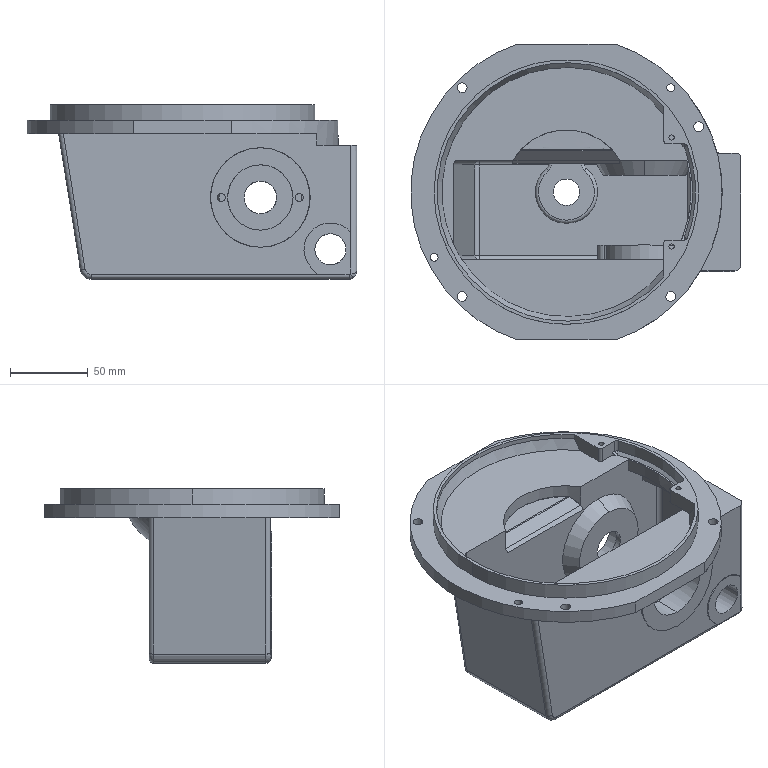CAM job | Mastercam | mm | 3 operations | part box 212 x 190 x 112
1. Contour (Ramp) | 6 - 21 平铣刀
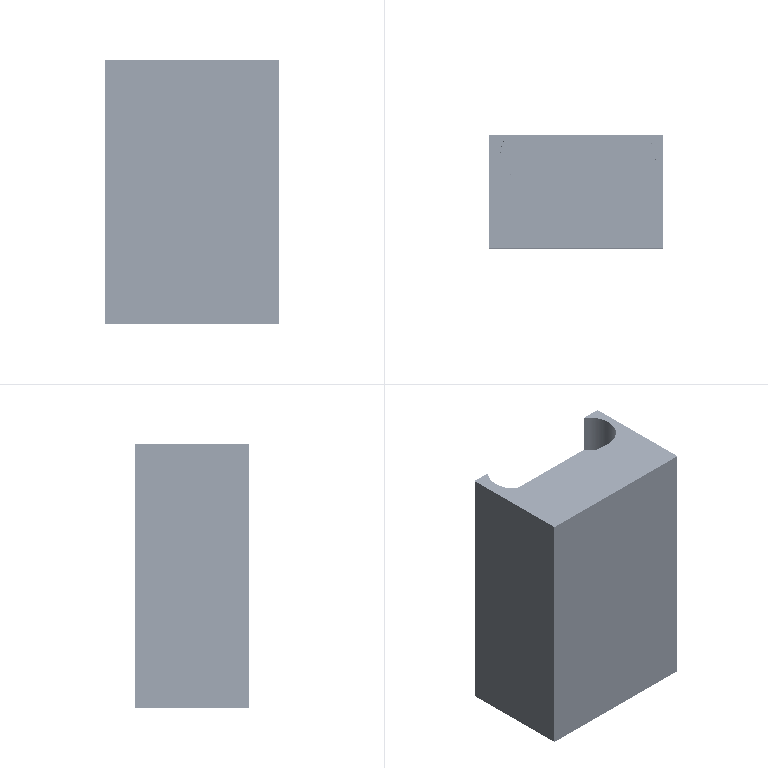2. Contour (Ramp) | 6 - 21 平铣刀
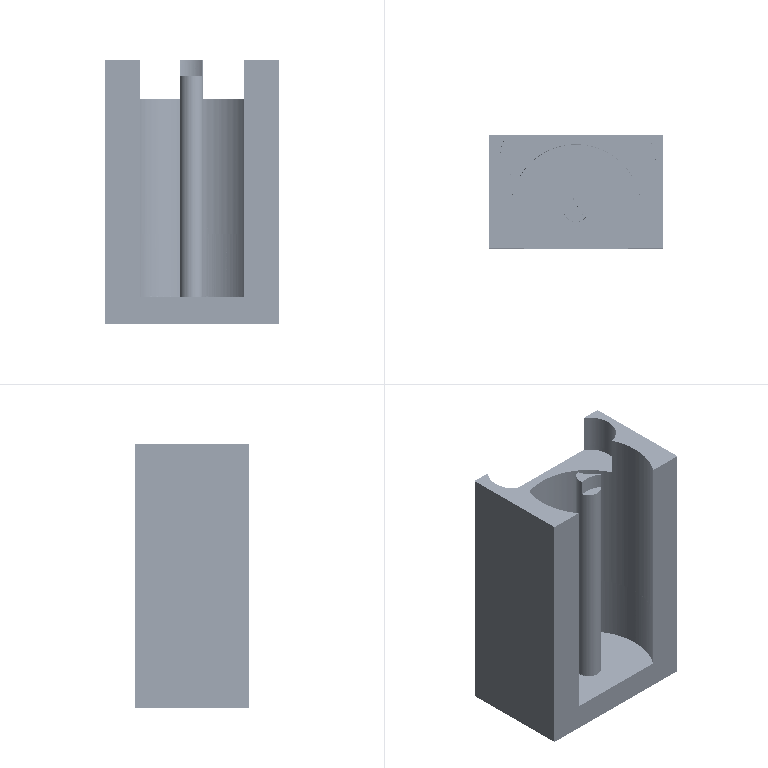3. Surface Finish Parallel | 2 - 10 平铣刀